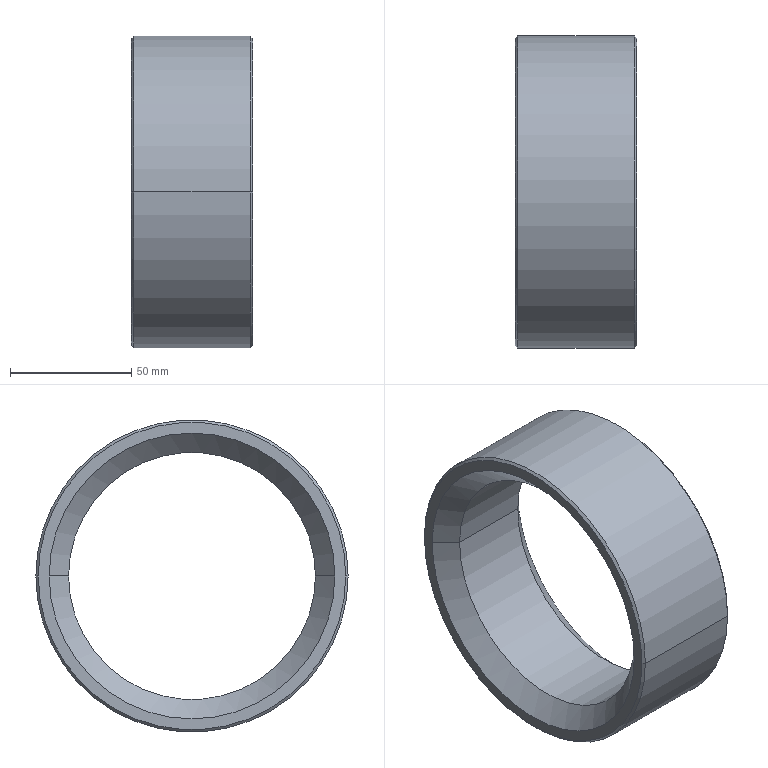Component | SolidWorks | 216OuterTube-1_SeatRing-1 | 1 solid | 14 faces | box 50 x 129 x 129 mm | volume 222943 mm3 | cone 8 | cylinder 4 | plane 2 | commonest cylinder face diameters 102 x2 129 x2 | material Alloy Steel
build123d program:
from build123d import *


with BuildPart() as part:
    # Model → Revolve1 (revolve)
    with BuildSketch(Plane.XY):
        Polygon((0.8417, 58.529), (0.8417, 63.029), (-0.1583, 64.029), (-48.158, 64.029), (-49.158, 63.029), (-49.158, 58.529), (-41.158, 50.529), (-7.158, 50.529), align=None)
    revolve(axis=Axis((2.022, -0.4715, 0), (-1, 0, 0)))


solid = part.part

# Placed as in the assembly
solid = solid.moved(Location((691.237, 0.4715, 0), (0, 0, 0)))
STEP:
#1=CARTESIAN_POINT('',(25.594,-2.008,0.));
#2=VERTEX_POINT('',#1);
#3=CARTESIAN_POINT('',(25.594,2.008,0.));
#4=VERTEX_POINT('',#3);
#5=CARTESIAN_POINT('',(25.594,-0.,0.));
#6=DIRECTION('',(1.,0.,0.));
#7=DIRECTION('',(0.,1.,0.));
#8=AXIS2_PLACEMENT_3D('',#5,#6,#7);
#9=CIRCLE('',#8,2.008);
#10=EDGE_CURVE('',#2,#4,#9,.T.);
#11=ORIENTED_EDGE('',*,*,#10,.F.);
#12=CARTESIAN_POINT('',(26.932,-2.008,0.));
#13=VERTEX_POINT('',#12);
#14=CARTESIAN_POINT('',(27.294,-2.008,0.));
#15=DIRECTION('',(1.,0.,0.));
#16=VECTOR('',#15,39.37);
#17=LINE('',#14,#16);
#18=EDGE_CURVE('',#2,#13,#17,.T.);
#19=ORIENTED_EDGE('',*,*,#18,.T.);
#20=CARTESIAN_POINT('',(26.932,2.008,0.));
#21=VERTEX_POINT('',#20);
#22=CARTESIAN_POINT('',(26.932,-0.,0.));
#23=DIRECTION('',(1.,0.,0.));
#24=DIRECTION('',(0.,1.,0.));
#25=AXIS2_PLACEMENT_3D('',#22,#23,#24);
#26=CIRCLE('',#25,2.008);
#27=EDGE_CURVE('',#13,#21,#26,.T.);
#28=ORIENTED_EDGE('',*,*,#27,.T.);
#29=CARTESIAN_POINT('',(27.294,2.008,0.));
#30=DIRECTION('',(1.,0.,0.));
#31=VECTOR('',#30,39.37);
#32=LINE('',#29,#31);
#33=EDGE_CURVE('',#4,#21,#32,.T.);
#34=ORIENTED_EDGE('',*,*,#33,.F.);
#35=EDGE_LOOP('',(#11,#19,#28,#34));
#36=FACE_OUTER_BOUND('',#35,.T.);
#37=CARTESIAN_POINT('',(27.294,0.,0.));
#38=DIRECTION('',(1.,0.,0.));
#39=DIRECTION('',(0.,1.,0.));
#40=AXIS2_PLACEMENT_3D('',#37,#38,#39);
#41=CYLINDRICAL_SURFACE('',#40,2.008);
#42=ADVANCED_FACE('',(#36),#41,.F.);
#43=ORIENTED_EDGE('',*,*,#10,.T.);
#44=CARTESIAN_POINT('',(25.279,2.323,0.));
#45=VERTEX_POINT('',#44);
#46=CARTESIAN_POINT('',(25.279,2.323,0.));
#47=DIRECTION('',(-0.7071,0.7071,0.));
#48=VECTOR('',#47,39.37);
#49=LINE('',#46,#48);
#50=EDGE_CURVE('',#4,#45,#49,.T.);
#51=ORIENTED_EDGE('',*,*,#50,.T.);
#52=CARTESIAN_POINT('',(25.279,-2.323,0.));
#53=VERTEX_POINT('',#52);
#54=CARTESIAN_POINT('',(25.279,-0.,0.));
#55=DIRECTION('',(1.,0.,0.));
#56=DIRECTION('',(0.,1.,0.));
#57=AXIS2_PLACEMENT_3D('',#54,#55,#56);
#58=CIRCLE('',#57,2.323);
#59=EDGE_CURVE('',#53,#45,#58,.T.);
#60=ORIENTED_EDGE('',*,*,#59,.F.);
#61=CARTESIAN_POINT('',(25.279,-2.323,0.));
#62=DIRECTION('',(-0.7071,-0.7071,0.));
#63=VECTOR('',#62,39.37);
#64=LINE('',#61,#63);
#65=EDGE_CURVE('',#2,#53,#64,.T.);
#66=ORIENTED_EDGE('',*,*,#65,.F.);
#67=EDGE_LOOP('',(#43,#51,#60,#66));
#68=FACE_OUTER_BOUND('',#67,.T.);
#69=CARTESIAN_POINT('',(25.279,-0.,0.));
#70=DIRECTION('',(-1.,-0.,0.));
#71=DIRECTION('',(0.,-1.,0.));
#72=AXIS2_PLACEMENT_3D('',#69,#70,#71);
#73=CONICAL_SURFACE('',#72,2.323,0.7854);
#74=ADVANCED_FACE('',(#68),#73,.F.);
#75=CARTESIAN_POINT('',(25.279,2.5,0.));
#76=VERTEX_POINT('',#75);
#77=CARTESIAN_POINT('',(25.279,-2.5,0.));
#78=VERTEX_POINT('',#77);
#79=CARTESIAN_POINT('',(25.279,-0.,0.));
#80=DIRECTION('',(1.,0.,0.));
#81=DIRECTION('',(0.,1.,0.));
#82=AXIS2_PLACEMENT_3D('',#79,#80,#81);
#83=CIRCLE('',#82,2.5);
#84=EDGE_CURVE('',#76,#78,#83,.T.);
#85=ORIENTED_EDGE('',*,*,#84,.T.);
#86=CARTESIAN_POINT('',(25.318,-2.539,0.));
#87=VERTEX_POINT('',#86);
#88=CARTESIAN_POINT('',(25.318,-2.539,0.));
#89=DIRECTION('',(0.7071,-0.7071,0.));
#90=VECTOR('',#89,39.37);
#91=LINE('',#88,#90);
#92=EDGE_CURVE('',#78,#87,#91,.T.);
#93=ORIENTED_EDGE('',*,*,#92,.T.);
#94=CARTESIAN_POINT('',(25.318,2.539,0.));
#95=VERTEX_POINT('',#94);
#96=CARTESIAN_POINT('',(25.318,-0.,0.));
#97=DIRECTION('',(1.,0.,0.));
#98=DIRECTION('',(0.,1.,0.));
#99=AXIS2_PLACEMENT_3D('',#96,#97,#98);
#100=CIRCLE('',#99,2.539);
#101=EDGE_CURVE('',#95,#87,#100,.T.);
#102=ORIENTED_EDGE('',*,*,#101,.F.);
#103=CARTESIAN_POINT('',(25.318,2.539,0.));
#104=DIRECTION('',(0.7071,0.7071,0.));
#105=VECTOR('',#104,39.37);
#106=LINE('',#103,#105);
#107=EDGE_CURVE('',#76,#95,#106,.T.);
#108=ORIENTED_EDGE('',*,*,#107,.F.);
#109=EDGE_LOOP('',(#85,#93,#102,#108));
#110=FACE_OUTER_BOUND('',#109,.T.);
#111=CARTESIAN_POINT('',(25.318,-0.,0.));
#112=DIRECTION('',(1.,0.,0.));
#113=DIRECTION('',(0.,1.,0.));
#114=AXIS2_PLACEMENT_3D('',#111,#112,#113);
#115=CONICAL_SURFACE('',#114,2.539,0.7854);
#116=ADVANCED_FACE('',(#110),#115,.T.);
#117=ORIENTED_EDGE('',*,*,#101,.T.);
#118=CARTESIAN_POINT('',(27.208,-2.539,0.));
#119=VERTEX_POINT('',#118);
#120=CARTESIAN_POINT('',(27.294,-2.539,0.));
#121=DIRECTION('',(1.,0.,0.));
#122=VECTOR('',#121,39.37);
#123=LINE('',#120,#122);
#124=EDGE_CURVE('',#87,#119,#123,.T.);
#125=ORIENTED_EDGE('',*,*,#124,.T.);
#126=CARTESIAN_POINT('',(27.208,2.539,0.));
#127=VERTEX_POINT('',#126);
#128=CARTESIAN_POINT('',(27.208,-0.,0.));
#129=DIRECTION('',(1.,0.,0.));
#130=DIRECTION('',(0.,1.,0.));
#131=AXIS2_PLACEMENT_3D('',#128,#129,#130);
#132=CIRCLE('',#131,2.539);
#133=EDGE_CURVE('',#127,#119,#132,.T.);
#134=ORIENTED_EDGE('',*,*,#133,.F.);
#135=CARTESIAN_POINT('',(27.294,2.539,0.));
#136=DIRECTION('',(1.,0.,0.));
#137=VECTOR('',#136,39.37);
#138=LINE('',#135,#137);
#139=EDGE_CURVE('',#95,#127,#138,.T.);
#140=ORIENTED_EDGE('',*,*,#139,.F.);
#141=EDGE_LOOP('',(#117,#125,#134,#140));
#142=FACE_OUTER_BOUND('',#141,.T.);
#143=CARTESIAN_POINT('',(27.294,0.,0.));
#144=DIRECTION('',(1.,0.,0.));
#145=DIRECTION('',(0.,1.,0.));
#146=AXIS2_PLACEMENT_3D('',#143,#144,#145);
#147=CYLINDRICAL_SURFACE('',#146,2.539);
#148=ADVANCED_FACE('',(#142),#147,.T.);
#149=CARTESIAN_POINT('',(27.247,2.5,0.));
#150=VERTEX_POINT('',#149);
#151=CARTESIAN_POINT('',(27.247,-2.5,0.));
#152=VERTEX_POINT('',#151);
#153=CARTESIAN_POINT('',(27.247,-0.,0.));
#154=DIRECTION('',(1.,0.,0.));
#155=DIRECTION('',(0.,1.,0.));
#156=AXIS2_PLACEMENT_3D('',#153,#154,#155);
#157=CIRCLE('',#156,2.5);
#158=EDGE_CURVE('',#150,#152,#157,.T.);
#159=ORIENTED_EDGE('',*,*,#158,.F.);
#160=CARTESIAN_POINT('',(27.247,2.5,0.));
#161=DIRECTION('',(-0.7071,0.7071,0.));
#162=VECTOR('',#161,39.37);
#163=LINE('',#160,#162);
#164=EDGE_CURVE('',#150,#127,#163,.T.);
#165=ORIENTED_EDGE('',*,*,#164,.T.);
#166=ORIENTED_EDGE('',*,*,#133,.T.);
#167=CARTESIAN_POINT('',(27.247,-2.5,0.));
#168=DIRECTION('',(-0.7071,-0.7071,0.));
#169=VECTOR('',#168,39.37);
#170=LINE('',#167,#169);
#171=EDGE_CURVE('',#152,#119,#170,.T.);
#172=ORIENTED_EDGE('',*,*,#171,.F.);
#173=EDGE_LOOP('',(#159,#165,#166,#172));
#174=FACE_OUTER_BOUND('',#173,.T.);
#175=CARTESIAN_POINT('',(27.247,-0.,0.));
#176=DIRECTION('',(-1.,-0.,0.));
#177=DIRECTION('',(0.,-1.,0.));
#178=AXIS2_PLACEMENT_3D('',#175,#176,#177);
#179=CONICAL_SURFACE('',#178,2.5,0.7854);
#180=ADVANCED_FACE('',(#174),#179,.T.);
#181=ORIENTED_EDGE('',*,*,#27,.F.);
#182=CARTESIAN_POINT('',(27.247,-2.323,0.));
#183=VERTEX_POINT('',#182);
#184=CARTESIAN_POINT('',(26.932,-2.008,0.));
#185=DIRECTION('',(0.7071,-0.7071,0.));
#186=VECTOR('',#185,39.37);
#187=LINE('',#184,#186);
#188=EDGE_CURVE('',#13,#183,#187,.T.);
#189=ORIENTED_EDGE('',*,*,#188,.T.);
#190=CARTESIAN_POINT('',(27.247,2.323,0.));
#191=VERTEX_POINT('',#190);
#192=CARTESIAN_POINT('',(27.247,-0.,0.));
#193=DIRECTION('',(1.,0.,0.));
#194=DIRECTION('',(0.,1.,0.));
#195=AXIS2_PLACEMENT_3D('',#192,#193,#194);
#196=CIRCLE('',#195,2.323);
#197=EDGE_CURVE('',#183,#191,#196,.T.);
#198=ORIENTED_EDGE('',*,*,#197,.T.);
#199=CARTESIAN_POINT('',(26.932,2.008,0.));
#200=DIRECTION('',(0.7071,0.7071,0.));
#201=VECTOR('',#200,39.37);
#202=LINE('',#199,#201);
#203=EDGE_CURVE('',#21,#191,#202,.T.);
#204=ORIENTED_EDGE('',*,*,#203,.F.);
#205=EDGE_LOOP('',(#181,#189,#198,#204));
#206=FACE_OUTER_BOUND('',#205,.T.);
#207=CARTESIAN_POINT('',(26.932,-0.,0.));
#208=DIRECTION('',(1.,0.,0.));
#209=DIRECTION('',(0.,1.,0.));
#210=AXIS2_PLACEMENT_3D('',#207,#208,#209);
#211=CONICAL_SURFACE('',#210,2.008,0.7854);
#212=ADVANCED_FACE('',(#206),#211,.F.);
#213=ORIENTED_EDGE('',*,*,#188,.F.);
#214=CARTESIAN_POINT('',(26.932,-0.,0.));
#215=DIRECTION('',(1.,0.,0.));
#216=DIRECTION('',(0.,1.,0.));
#217=AXIS2_PLACEMENT_3D('',#214,#215,#216);
#218=CIRCLE('',#217,2.008);
#219=EDGE_CURVE('',#21,#13,#218,.T.);
#220=ORIENTED_EDGE('',*,*,#219,.F.);
#221=ORIENTED_EDGE('',*,*,#203,.T.);
#222=CARTESIAN_POINT('',(27.247,-0.,0.));
#223=DIRECTION('',(1.,0.,0.));
#224=DIRECTION('',(0.,1.,0.));
#225=AXIS2_PLACEMENT_3D('',#222,#223,#224);
#226=CIRCLE('',#225,2.323);
#227=EDGE_CURVE('',#191,#183,#226,.T.);
#228=ORIENTED_EDGE('',*,*,#227,.T.);
#229=EDGE_LOOP('',(#213,#220,#221,#228));
#230=FACE_OUTER_BOUND('',#229,.T.);
#231=CARTESIAN_POINT('',(26.932,-0.,0.));
#232=DIRECTION('',(1.,0.,0.));
#233=DIRECTION('',(0.,1.,0.));
#234=AXIS2_PLACEMENT_3D('',#231,#232,#233);
#235=CONICAL_SURFACE('',#234,2.008,0.7854);
#236=ADVANCED_FACE('',(#230),#235,.F.);
#237=CARTESIAN_POINT('',(27.247,-0.,0.));
#238=DIRECTION('',(1.,0.,0.));
#239=DIRECTION('',(0.,1.,0.));
#240=AXIS2_PLACEMENT_3D('',#237,#238,#239);
#241=CIRCLE('',#240,2.5);
#242=EDGE_CURVE('',#152,#150,#241,.T.);
#243=ORIENTED_EDGE('',*,*,#242,.T.);
#244=ORIENTED_EDGE('',*,*,#158,.T.);
#245=EDGE_LOOP('',(#243,#244));
#246=FACE_OUTER_BOUND('',#245,.T.);
#247=ORIENTED_EDGE('',*,*,#227,.F.);
#248=ORIENTED_EDGE('',*,*,#197,.F.);
#249=EDGE_LOOP('',(#247,#248));
#250=FACE_BOUND('',#249,.T.);
#251=CARTESIAN_POINT('',(27.247,2.323,0.));
#252=DIRECTION('',(1.,0.,0.));
#253=DIRECTION('',(-0.,1.,0.));
#254=AXIS2_PLACEMENT_3D('',#251,#252,#253);
#255=PLANE('',#254);
#256=ADVANCED_FACE('',(#246,#250),#255,.T.);
#257=ORIENTED_EDGE('',*,*,#164,.F.);
#258=ORIENTED_EDGE('',*,*,#242,.F.);
#259=ORIENTED_EDGE('',*,*,#171,.T.);
#260=CARTESIAN_POINT('',(27.208,-0.,0.));
#261=DIRECTION('',(1.,0.,0.));
#262=DIRECTION('',(0.,1.,0.));
#263=AXIS2_PLACEMENT_3D('',#260,#261,#262);
#264=CIRCLE('',#263,2.539);
#265=EDGE_CURVE('',#119,#127,#264,.T.);
#266=ORIENTED_EDGE('',*,*,#265,.T.);
#267=EDGE_LOOP('',(#257,#258,#259,#266));
#268=FACE_OUTER_BOUND('',#267,.T.);
#269=CARTESIAN_POINT('',(27.247,-0.,0.));
#270=DIRECTION('',(-1.,-0.,0.));
#271=DIRECTION('',(0.,-1.,0.));
#272=AXIS2_PLACEMENT_3D('',#269,#270,#271);
#273=CONICAL_SURFACE('',#272,2.5,0.7854);
#274=ADVANCED_FACE('',(#268),#273,.T.);
#275=ORIENTED_EDGE('',*,*,#124,.F.);
#276=CARTESIAN_POINT('',(25.318,-0.,0.));
#277=DIRECTION('',(1.,0.,0.));
#278=DIRECTION('',(0.,1.,0.));
#279=AXIS2_PLACEMENT_3D('',#276,#277,#278);
#280=CIRCLE('',#279,2.539);
#281=EDGE_CURVE('',#87,#95,#280,.T.);
#282=ORIENTED_EDGE('',*,*,#281,.T.);
#283=ORIENTED_EDGE('',*,*,#139,.T.);
#284=ORIENTED_EDGE('',*,*,#265,.F.);
#285=EDGE_LOOP('',(#275,#282,#283,#284));
#286=FACE_OUTER_BOUND('',#285,.T.);
#287=CARTESIAN_POINT('',(27.294,0.,0.));
#288=DIRECTION('',(1.,0.,0.));
#289=DIRECTION('',(0.,1.,0.));
#290=AXIS2_PLACEMENT_3D('',#287,#288,#289);
#291=CYLINDRICAL_SURFACE('',#290,2.539);
#292=ADVANCED_FACE('',(#286),#291,.T.);
#293=ORIENTED_EDGE('',*,*,#92,.F.);
#294=CARTESIAN_POINT('',(25.279,-0.,0.));
#295=DIRECTION('',(1.,0.,0.));
#296=DIRECTION('',(0.,1.,0.));
#297=AXIS2_PLACEMENT_3D('',#294,#295,#296);
#298=CIRCLE('',#297,2.5);
#299=EDGE_CURVE('',#78,#76,#298,.T.);
#300=ORIENTED_EDGE('',*,*,#299,.T.);
#301=ORIENTED_EDGE('',*,*,#107,.T.);
#302=ORIENTED_EDGE('',*,*,#281,.F.);
#303=EDGE_LOOP('',(#293,#300,#301,#302));
#304=FACE_OUTER_BOUND('',#303,.T.);
#305=CARTESIAN_POINT('',(25.318,-0.,0.));
#306=DIRECTION('',(1.,0.,0.));
#307=DIRECTION('',(0.,1.,0.));
#308=AXIS2_PLACEMENT_3D('',#305,#306,#307);
#309=CONICAL_SURFACE('',#308,2.539,0.7854);
#310=ADVANCED_FACE('',(#304),#309,.T.);
#311=ORIENTED_EDGE('',*,*,#59,.T.);
#312=CARTESIAN_POINT('',(25.279,-0.,0.));
#313=DIRECTION('',(1.,0.,0.));
#314=DIRECTION('',(0.,1.,0.));
#315=AXIS2_PLACEMENT_3D('',#312,#313,#314);
#316=CIRCLE('',#315,2.323);
#317=EDGE_CURVE('',#45,#53,#316,.T.);
#318=ORIENTED_EDGE('',*,*,#317,.T.);
#319=EDGE_LOOP('',(#311,#318));
#320=FACE_BOUND('',#319,.T.);
#321=ORIENTED_EDGE('',*,*,#84,.F.);
#322=ORIENTED_EDGE('',*,*,#299,.F.);
#323=EDGE_LOOP('',(#321,#322));
#324=FACE_OUTER_BOUND('',#323,.T.);
#325=CARTESIAN_POINT('',(25.279,2.5,0.));
#326=DIRECTION('',(-1.,-0.,0.));
#327=DIRECTION('',(0.,-1.,0.));
#328=AXIS2_PLACEMENT_3D('',#325,#326,#327);
#329=PLANE('',#328);
#330=ADVANCED_FACE('',(#320,#324),#329,.T.);
#331=ORIENTED_EDGE('',*,*,#50,.F.);
#332=CARTESIAN_POINT('',(25.594,-0.,0.));
#333=DIRECTION('',(1.,0.,0.));
#334=DIRECTION('',(0.,1.,0.));
#335=AXIS2_PLACEMENT_3D('',#332,#333,#334);
#336=CIRCLE('',#335,2.008);
#337=EDGE_CURVE('',#4,#2,#336,.T.);
#338=ORIENTED_EDGE('',*,*,#337,.T.);
#339=ORIENTED_EDGE('',*,*,#65,.T.);
#340=ORIENTED_EDGE('',*,*,#317,.F.);
#341=EDGE_LOOP('',(#331,#338,#339,#340));
#342=FACE_OUTER_BOUND('',#341,.T.);
#343=CARTESIAN_POINT('',(25.279,-0.,0.));
#344=DIRECTION('',(-1.,-0.,0.));
#345=DIRECTION('',(0.,-1.,0.));
#346=AXIS2_PLACEMENT_3D('',#343,#344,#345);
#347=CONICAL_SURFACE('',#346,2.323,0.7854);
#348=ADVANCED_FACE('',(#342),#347,.F.);
#349=ORIENTED_EDGE('',*,*,#18,.F.);
#350=ORIENTED_EDGE('',*,*,#337,.F.);
#351=ORIENTED_EDGE('',*,*,#33,.T.);
#352=ORIENTED_EDGE('',*,*,#219,.T.);
#353=EDGE_LOOP('',(#349,#350,#351,#352));
#354=FACE_OUTER_BOUND('',#353,.T.);
#355=CARTESIAN_POINT('',(27.294,0.,0.));
#356=DIRECTION('',(1.,0.,0.));
#357=DIRECTION('',(0.,1.,0.));
#358=AXIS2_PLACEMENT_3D('',#355,#356,#357);
#359=CYLINDRICAL_SURFACE('',#358,2.008);
#360=ADVANCED_FACE('',(#354),#359,.F.);
#361=CLOSED_SHELL('',(#42,#74,#116,#148,#180,#212,#236,#256,#274,#292,#310,#330,#348,#360));
#362=MANIFOLD_SOLID_BREP('',#361);
#363=CARTESIAN_POINT('',(0.,0.,0.));
#364=DIRECTION('',(0.,0.,1.));
#365=DIRECTION('',(1.,0.,0.));
#366=AXIS2_PLACEMENT_3D('',#363,#364,#365);
#367=(LENGTH_UNIT()NAMED_UNIT(*)SI_UNIT($,.METRE.));
#368=LENGTH_MEASURE_WITH_UNIT(LENGTH_MEASURE(0.0254),#367);
#369=DIMENSIONAL_EXPONENTS(1.,0.,0.,0.,0.,0.,0.);
#370=(CONVERSION_BASED_UNIT('',#368)LENGTH_UNIT()NAMED_UNIT(#369));
#371=UNCERTAINTY_MEASURE_WITH_UNIT(LENGTH_MEASURE(0.00001),#370,'','');
#372=(NAMED_UNIT(*)PLANE_ANGLE_UNIT()SI_UNIT($,.RADIAN.));
#373=(NAMED_UNIT(*)SI_UNIT($,.STERADIAN.)SOLID_ANGLE_UNIT());
#374=(GEOMETRIC_REPRESENTATION_CONTEXT(3)GLOBAL_UNCERTAINTY_ASSIGNED_CONTEXT((#371))GLOBAL_UNIT_ASSIGNED_CONTEXT((#370,#372,#373))REPRESENTATION_CONTEXT('',''));
#375=ADVANCED_BREP_SHAPE_REPRESENTATION('',(#362,#366),#374);
#376=COLOUR_RGB('',0.7922,0.8196,0.9333);
#377=FILL_AREA_STYLE_COLOUR('',#376);
#378=FILL_AREA_STYLE('',(#377));
#379=SURFACE_STYLE_FILL_AREA(#378);
#380=SURFACE_SIDE_STYLE('',(#379));
#381=SURFACE_STYLE_USAGE(.BOTH.,#380);
#382=PRESENTATION_STYLE_ASSIGNMENT((#381));
#383=STYLED_ITEM('',(#382),#362);
#384=PRESENTATION_LAYER_ASSIGNMENT('','',(#383));
#385=(LENGTH_UNIT()NAMED_UNIT(*)SI_UNIT($,.METRE.));
#386=LENGTH_MEASURE_WITH_UNIT(LENGTH_MEASURE(0.0254),#385);
#387=DIMENSIONAL_EXPONENTS(1.,0.,0.,0.,0.,0.,0.);
#388=(CONVERSION_BASED_UNIT('',#386)LENGTH_UNIT()NAMED_UNIT(#387));
#389=UNCERTAINTY_MEASURE_WITH_UNIT(LENGTH_MEASURE(0.00001),#388,'','');
#390=(NAMED_UNIT(*)PLANE_ANGLE_UNIT()SI_UNIT($,.RADIAN.));
#391=(NAMED_UNIT(*)SI_UNIT($,.STERADIAN.)SOLID_ANGLE_UNIT());
#392=(GEOMETRIC_REPRESENTATION_CONTEXT(3)GLOBAL_UNCERTAINTY_ASSIGNED_CONTEXT((#389))GLOBAL_UNIT_ASSIGNED_CONTEXT((#388,#390,#391))REPRESENTATION_CONTEXT('',''));
#393=MECHANICAL_DESIGN_GEOMETRIC_PRESENTATION_REPRESENTATION('',(#383),#392);